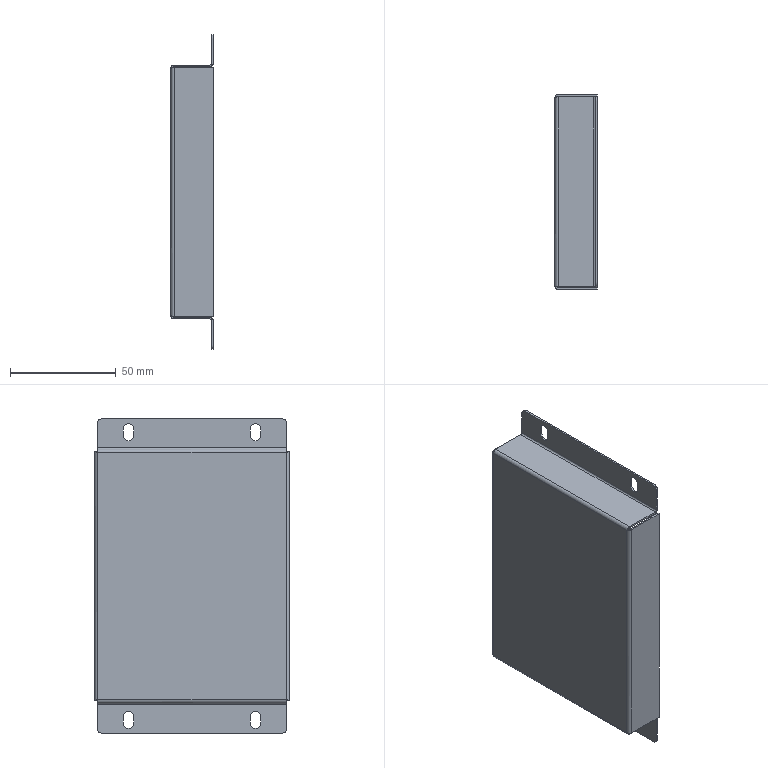Component | SolidWorks | CoverPlate.1-1 | 1 solid | 78 faces | volume 16889 mm3 | plane 42 | cylinder 28 | spline 8 | commonest cylinder face diameters 5 x12 3.073 x6 1.473 x6 4 x4